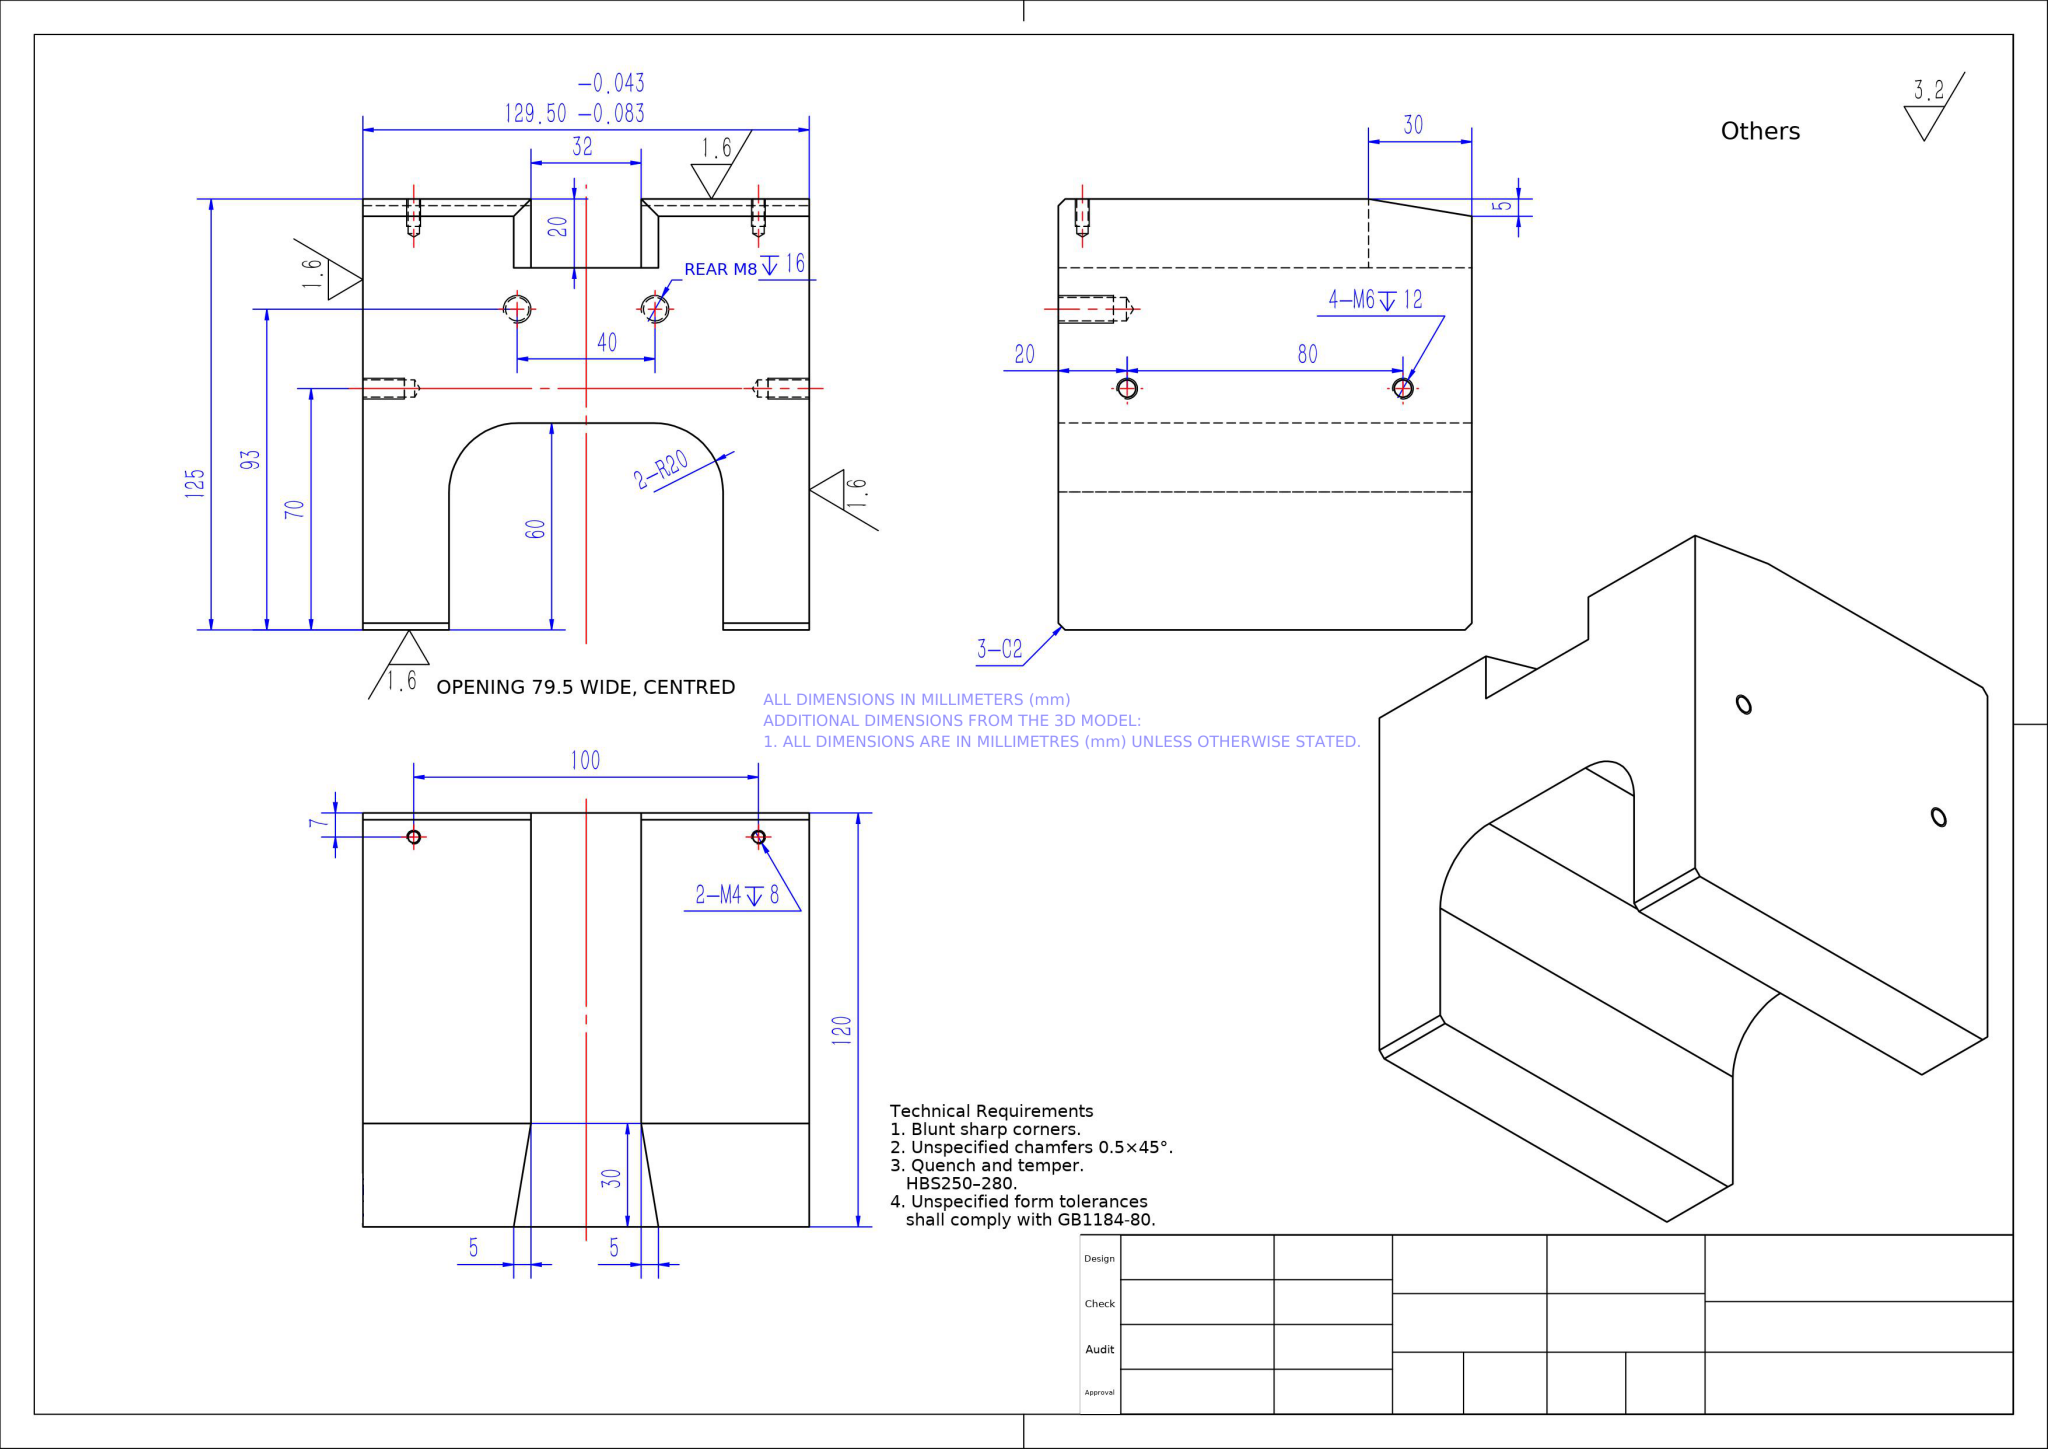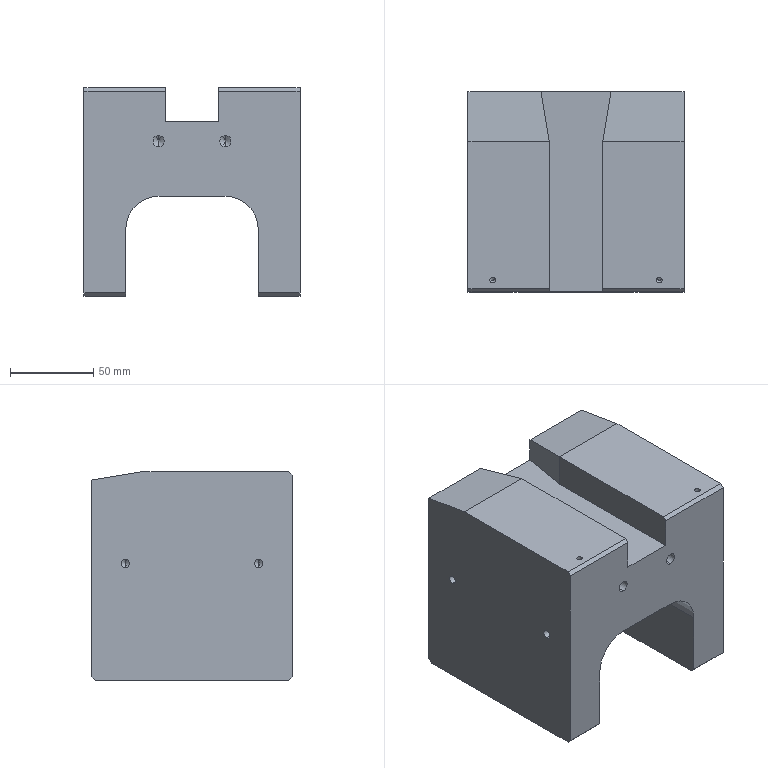Part | NX | mm | Dual-Pedestal Arched Mounting Bracket | 1 solid | 58 faces | box 129.5 x 120 x 125 mm | volume 1300814 mm3 | plane 24 | cylinder 18 | cone 16 | commonest cylinder face diameters 5 x8 3.3 x4 6.8 x4 40 x2